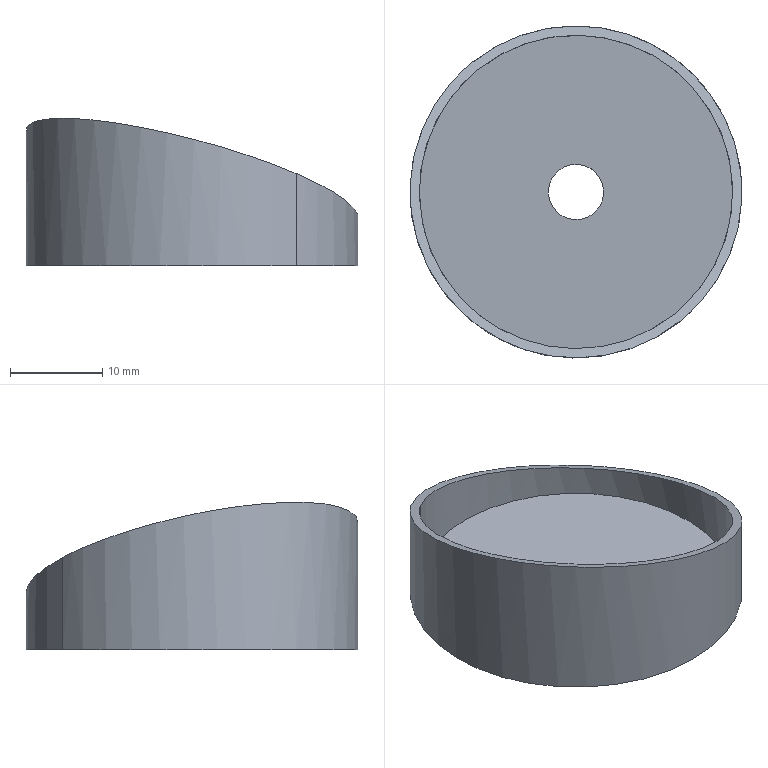Component | SolidWorks | GRingCam-8 | 1 solid | 9 faces | box 36 x 36 x 16 mm | volume 1979 mm3 | cylinder 6 | plane 3 | commonest cylinder face diameters 6 x2 36 x2 34 x2
build123d program:
from build123d import *

# Parameters (mm, degrees)
SKETCH2_R           = 18
SKETCH2_R_2         = 17
BOSS_EXTRUDE1_DEPTH = 8
CUT_EXTRUDE1_DEPTH  = 27
BOSS_EXTRUDE2_START = -1
SKETCH4_R           = 18
SKETCH4_R_2         = 3
BOSS_EXTRUDE2_DEPTH = 1


with BuildPart() as part:
    # Sketch2 → Boss-Extrude1 (new, symmetric)
    with BuildSketch(Plane(origin=(0, 0, 0), x_dir=(1, 0, 0), z_dir=(0, 1, 0))):
        with Locations(Location((0, 0, 0), (0, 0, 270))):
            Circle(SKETCH2_R)
        with Locations(Location((0, 0, 0), (0, 0, 270))):
            Circle(SKETCH2_R_2, mode=Mode.SUBTRACT)
    extrude(amount=BOSS_EXTRUDE1_DEPTH, both=True)

    # Sketch3 → Cut-Extrude1 (cut, symmetric)
    with BuildSketch(Plane.XY):
        Polygon((-24.457, 9.582), (-18, -4), (18, 8), align=None)
    extrude(amount=CUT_EXTRUDE1_DEPTH, both=True, mode=Mode.SUBTRACT)

    # Sketch4 → Boss-Extrude2 (add)
    with BuildSketch(Plane.XZ.offset(8).offset(BOSS_EXTRUDE2_START)):
        with Locations(Location((0, 0, 0), (0, 0, 180))):
            Circle(SKETCH4_R)
        with Locations(Location((0, 0, 0), (0, 0, 270))):
            Circle(SKETCH4_R_2, mode=Mode.SUBTRACT)
    extrude(amount=BOSS_EXTRUDE2_DEPTH)


solid = part.part

# Placed as in the assembly
solid = solid.moved(Location((-15.928, -22.2, 125), (-90, -38.823, 179.998)))
STEP:
#1=COLOUR_RGB('',0.7922,0.8196,0.9333);
#2=FILL_AREA_STYLE_COLOUR('',#1);
#3=FILL_AREA_STYLE('',(#2));
#4=SURFACE_STYLE_FILL_AREA(#3);
#5=SURFACE_SIDE_STYLE('',(#4));
#6=SURFACE_STYLE_USAGE(.BOTH.,#5);
#7=PRESENTATION_STYLE_ASSIGNMENT((#6));
#8=CARTESIAN_POINT('',(-0.7011,-0.782,4.646));
#9=VERTEX_POINT('',#8);
#10=CARTESIAN_POINT('',(-0.553,-0.966,4.646));
#11=VERTEX_POINT('',#10);
#12=CARTESIAN_POINT('',(-0.6271,-0.874,4.646));
#13=DIRECTION('',(0.,0.,-1.));
#14=DIRECTION('',(0.6269,-0.7791,0.));
#15=AXIS2_PLACEMENT_3D('',#12,#13,#14);
#16=CIRCLE('',#15,0.1181);
#17=EDGE_CURVE('',#9,#11,#16,.T.);
#18=ORIENTED_EDGE('',*,*,#17,.F.);
#19=CARTESIAN_POINT('',(-0.7011,-0.782,4.606));
#20=VERTEX_POINT('',#19);
#21=CARTESIAN_POINT('',(-0.7011,-0.782,4.646));
#22=DIRECTION('',(0.,0.,-1.));
#23=VECTOR('',#22,39.37);
#24=LINE('',#21,#23);
#25=EDGE_CURVE('',#9,#20,#24,.T.);
#26=ORIENTED_EDGE('',*,*,#25,.T.);
#27=CARTESIAN_POINT('',(-0.553,-0.966,4.606));
#28=VERTEX_POINT('',#27);
#29=CARTESIAN_POINT('',(-0.6271,-0.874,4.606));
#30=DIRECTION('',(0.,0.,-1.));
#31=DIRECTION('',(0.6269,-0.7791,0.));
#32=AXIS2_PLACEMENT_3D('',#29,#30,#31);
#33=CIRCLE('',#32,0.1181);
#34=EDGE_CURVE('',#20,#28,#33,.T.);
#35=ORIENTED_EDGE('',*,*,#34,.T.);
#36=CARTESIAN_POINT('',(-0.553,-0.966,4.646));
#37=DIRECTION('',(0.,0.,-1.));
#38=VECTOR('',#37,39.37);
#39=LINE('',#36,#38);
#40=EDGE_CURVE('',#11,#28,#39,.T.);
#41=ORIENTED_EDGE('',*,*,#40,.F.);
#42=EDGE_LOOP('',(#18,#26,#35,#41));
#43=FACE_OUTER_BOUND('',#42,.T.);
#44=CARTESIAN_POINT('',(-0.6271,-0.874,4.646));
#45=DIRECTION('',(0.,0.,-1.));
#46=DIRECTION('',(0.6269,-0.7791,0.));
#47=AXIS2_PLACEMENT_3D('',#44,#45,#46);
#48=CYLINDRICAL_SURFACE('',#47,0.1181);
#49=ADVANCED_FACE('',(#43),#48,.F.);
#50=CARTESIAN_POINT('',(-0.1828,-1.426,5.));
#51=VERTEX_POINT('',#50);
#52=CARTESIAN_POINT('',(-1.071,-0.3219,5.));
#53=VERTEX_POINT('',#52);
#54=CARTESIAN_POINT('',(-0.1828,-1.426,5.));
#55=CARTESIAN_POINT('',(-1.287,-2.315,5.472));
#56=CARTESIAN_POINT('',(-2.176,-1.21,5.472));
#57=CARTESIAN_POINT('',(-1.071,-0.3219,5.));
#58=(BOUNDED_CURVE()B_SPLINE_CURVE(3,(#54,#55,#56,#57),.UNSPECIFIED.,.F.,.T.)B_SPLINE_CURVE_WITH_KNOTS((4,4),(1.571,4.712),.UNSPECIFIED.)CURVE()GEOMETRIC_REPRESENTATION_ITEM()RATIONAL_B_SPLINE_CURVE((1.,0.3333,0.3333,1.))REPRESENTATION_ITEM(''));
#59=EDGE_CURVE('',#51,#53,#58,.T.);
#60=ORIENTED_EDGE('',*,*,#59,.T.);
#61=CARTESIAN_POINT('',(-1.071,-0.3219,4.606));
#62=VERTEX_POINT('',#61);
#63=CARTESIAN_POINT('',(-1.071,-0.3219,5.236));
#64=DIRECTION('',(0.,0.,-1.));
#65=VECTOR('',#64,39.37);
#66=LINE('',#63,#65);
#67=EDGE_CURVE('',#53,#62,#66,.T.);
#68=ORIENTED_EDGE('',*,*,#67,.T.);
#69=CARTESIAN_POINT('',(-0.1828,-1.426,4.606));
#70=VERTEX_POINT('',#69);
#71=CARTESIAN_POINT('',(-0.6271,-0.874,4.606));
#72=DIRECTION('',(-0.,-0.,1.));
#73=DIRECTION('',(-0.6269,0.7791,0.));
#74=AXIS2_PLACEMENT_3D('',#71,#72,#73);
#75=CIRCLE('',#74,0.7087);
#76=EDGE_CURVE('',#62,#70,#75,.T.);
#77=ORIENTED_EDGE('',*,*,#76,.T.);
#78=CARTESIAN_POINT('',(-0.1828,-1.426,5.236));
#79=DIRECTION('',(0.,0.,-1.));
#80=VECTOR('',#79,39.37);
#81=LINE('',#78,#80);
#82=EDGE_CURVE('',#51,#70,#81,.T.);
#83=ORIENTED_EDGE('',*,*,#82,.F.);
#84=EDGE_LOOP('',(#60,#68,#77,#83));
#85=FACE_OUTER_BOUND('',#84,.T.);
#86=CARTESIAN_POINT('',(-0.6271,-0.874,5.236));
#87=DIRECTION('',(0.,0.,-1.));
#88=DIRECTION('',(0.6269,-0.7791,0.));
#89=AXIS2_PLACEMENT_3D('',#86,#87,#88);
#90=CYLINDRICAL_SURFACE('',#89,0.7087);
#91=ADVANCED_FACE('',(#85),#90,.T.);
#92=CARTESIAN_POINT('',(-1.047,-0.3526,5.));
#93=VERTEX_POINT('',#92);
#94=CARTESIAN_POINT('',(-0.2075,-1.395,5.));
#95=VERTEX_POINT('',#94);
#96=CARTESIAN_POINT('',(-1.047,-0.3526,5.));
#97=CARTESIAN_POINT('',(-0.003795,0.4866,4.554));
#98=CARTESIAN_POINT('',(0.8354,-0.5563,4.554));
#99=CARTESIAN_POINT('',(-0.2075,-1.395,5.));
#100=(BOUNDED_CURVE()B_SPLINE_CURVE(3,(#96,#97,#98,#99),.UNSPECIFIED.,.F.,.F.)B_SPLINE_CURVE_WITH_KNOTS((4,4),(4.712,7.854),.UNSPECIFIED.)CURVE()GEOMETRIC_REPRESENTATION_ITEM()RATIONAL_B_SPLINE_CURVE((1.,0.3333,0.3333,1.))REPRESENTATION_ITEM(''));
#101=EDGE_CURVE('',#93,#95,#100,.T.);
#102=ORIENTED_EDGE('',*,*,#101,.F.);
#103=CARTESIAN_POINT('',(-1.047,-0.3526,4.646));
#104=VERTEX_POINT('',#103);
#105=CARTESIAN_POINT('',(-1.047,-0.3526,5.236));
#106=DIRECTION('',(0.,0.,-1.));
#107=VECTOR('',#106,39.37);
#108=LINE('',#105,#107);
#109=EDGE_CURVE('',#93,#104,#108,.T.);
#110=ORIENTED_EDGE('',*,*,#109,.T.);
#111=CARTESIAN_POINT('',(-0.2075,-1.395,4.646));
#112=VERTEX_POINT('',#111);
#113=CARTESIAN_POINT('',(-0.6271,-0.874,4.646));
#114=DIRECTION('',(0.,0.,-1.));
#115=DIRECTION('',(0.6269,-0.7791,0.));
#116=AXIS2_PLACEMENT_3D('',#113,#114,#115);
#117=CIRCLE('',#116,0.6693);
#118=EDGE_CURVE('',#104,#112,#117,.T.);
#119=ORIENTED_EDGE('',*,*,#118,.T.);
#120=CARTESIAN_POINT('',(-0.2075,-1.395,5.236));
#121=DIRECTION('',(0.,0.,-1.));
#122=VECTOR('',#121,39.37);
#123=LINE('',#120,#122);
#124=EDGE_CURVE('',#95,#112,#123,.T.);
#125=ORIENTED_EDGE('',*,*,#124,.F.);
#126=EDGE_LOOP('',(#102,#110,#119,#125));
#127=FACE_OUTER_BOUND('',#126,.T.);
#128=CARTESIAN_POINT('',(-0.6271,-0.874,5.236));
#129=DIRECTION('',(0.,0.,-1.));
#130=DIRECTION('',(0.6269,-0.7791,0.));
#131=AXIS2_PLACEMENT_3D('',#128,#129,#130);
#132=CYLINDRICAL_SURFACE('',#131,0.6693);
#133=ADVANCED_FACE('',(#127),#132,.F.);
#134=ORIENTED_EDGE('',*,*,#109,.F.);
#135=CARTESIAN_POINT('',(-0.2075,-1.395,5.));
#136=CARTESIAN_POINT('',(-1.25,-2.235,5.446));
#137=CARTESIAN_POINT('',(-2.09,-1.192,5.446));
#138=CARTESIAN_POINT('',(-1.047,-0.3526,5.));
#139=(BOUNDED_CURVE()B_SPLINE_CURVE(3,(#135,#136,#137,#138),.UNSPECIFIED.,.F.,.T.)B_SPLINE_CURVE_WITH_KNOTS((4,4),(1.571,4.712),.UNSPECIFIED.)CURVE()GEOMETRIC_REPRESENTATION_ITEM()RATIONAL_B_SPLINE_CURVE((1.,0.3333,0.3333,1.))REPRESENTATION_ITEM(''));
#140=EDGE_CURVE('',#95,#93,#139,.T.);
#141=ORIENTED_EDGE('',*,*,#140,.F.);
#142=ORIENTED_EDGE('',*,*,#124,.T.);
#143=CARTESIAN_POINT('',(-0.6271,-0.874,4.646));
#144=DIRECTION('',(0.,0.,-1.));
#145=DIRECTION('',(0.6269,-0.7791,0.));
#146=AXIS2_PLACEMENT_3D('',#143,#144,#145);
#147=CIRCLE('',#146,0.6693);
#148=EDGE_CURVE('',#112,#104,#147,.T.);
#149=ORIENTED_EDGE('',*,*,#148,.T.);
#150=EDGE_LOOP('',(#134,#141,#142,#149));
#151=FACE_OUTER_BOUND('',#150,.T.);
#152=CARTESIAN_POINT('',(-0.6271,-0.874,5.236));
#153=DIRECTION('',(0.,0.,-1.));
#154=DIRECTION('',(0.6269,-0.7791,0.));
#155=AXIS2_PLACEMENT_3D('',#152,#153,#154);
#156=CYLINDRICAL_SURFACE('',#155,0.6693);
#157=ADVANCED_FACE('',(#151),#156,.F.);
#158=CARTESIAN_POINT('',(-0.6271,-0.874,4.606));
#159=DIRECTION('',(-0.,-0.,1.));
#160=DIRECTION('',(-0.6269,0.7791,0.));
#161=AXIS2_PLACEMENT_3D('',#158,#159,#160);
#162=CIRCLE('',#161,0.7087);
#163=EDGE_CURVE('',#70,#62,#162,.T.);
#164=ORIENTED_EDGE('',*,*,#163,.F.);
#165=ORIENTED_EDGE('',*,*,#76,.F.);
#166=EDGE_LOOP('',(#164,#165));
#167=FACE_OUTER_BOUND('',#166,.T.);
#168=CARTESIAN_POINT('',(-0.6271,-0.874,4.606));
#169=DIRECTION('',(0.,0.,-1.));
#170=DIRECTION('',(0.6269,-0.7791,0.));
#171=AXIS2_PLACEMENT_3D('',#168,#169,#170);
#172=CIRCLE('',#171,0.1181);
#173=EDGE_CURVE('',#28,#20,#172,.T.);
#174=ORIENTED_EDGE('',*,*,#173,.F.);
#175=ORIENTED_EDGE('',*,*,#34,.F.);
#176=EDGE_LOOP('',(#174,#175));
#177=FACE_BOUND('',#176,.T.);
#178=CARTESIAN_POINT('',(-0.6271,-0.874,4.606));
#179=DIRECTION('',(-0.,-0.,1.));
#180=DIRECTION('',(-0.6269,0.7791,0.));
#181=AXIS2_PLACEMENT_3D('',#178,#179,#180);
#182=PLANE('',#181);
#183=ADVANCED_FACE('',(#167,#177),#182,.F.);
#184=ORIENTED_EDGE('',*,*,#67,.F.);
#185=CARTESIAN_POINT('',(-1.071,-0.3219,5.));
#186=CARTESIAN_POINT('',(0.03287,0.5666,4.528));
#187=CARTESIAN_POINT('',(0.9214,-0.5376,4.528));
#188=CARTESIAN_POINT('',(-0.1828,-1.426,5.));
#189=(BOUNDED_CURVE()B_SPLINE_CURVE(3,(#185,#186,#187,#188),.UNSPECIFIED.,.F.,.F.)B_SPLINE_CURVE_WITH_KNOTS((4,4),(4.712,7.854),.UNSPECIFIED.)CURVE()GEOMETRIC_REPRESENTATION_ITEM()RATIONAL_B_SPLINE_CURVE((1.,0.3333,0.3333,1.))REPRESENTATION_ITEM(''));
#190=EDGE_CURVE('',#53,#51,#189,.T.);
#191=ORIENTED_EDGE('',*,*,#190,.T.);
#192=ORIENTED_EDGE('',*,*,#82,.T.);
#193=ORIENTED_EDGE('',*,*,#163,.T.);
#194=EDGE_LOOP('',(#184,#191,#192,#193));
#195=FACE_OUTER_BOUND('',#194,.T.);
#196=CARTESIAN_POINT('',(-0.6271,-0.874,5.236));
#197=DIRECTION('',(0.,0.,-1.));
#198=DIRECTION('',(0.6269,-0.7791,0.));
#199=AXIS2_PLACEMENT_3D('',#196,#197,#198);
#200=CYLINDRICAL_SURFACE('',#199,0.7087);
#201=ADVANCED_FACE('',(#195),#200,.T.);
#202=ORIENTED_EDGE('',*,*,#140,.T.);
#203=ORIENTED_EDGE('',*,*,#101,.T.);
#204=EDGE_LOOP('',(#202,#203));
#205=FACE_BOUND('',#204,.T.);
#206=ORIENTED_EDGE('',*,*,#59,.F.);
#207=ORIENTED_EDGE('',*,*,#190,.F.);
#208=EDGE_LOOP('',(#206,#207));
#209=FACE_OUTER_BOUND('',#208,.T.);
#210=CARTESIAN_POINT('',(0.5914,-1.258,4.764));
#211=DIRECTION('',(-0.2464,-0.1982,-0.9487));
#212=DIRECTION('',(-0.7391,-0.5947,0.3162));
#213=AXIS2_PLACEMENT_3D('',#210,#211,#212);
#214=PLANE('',#213);
#215=ADVANCED_FACE('',(#205,#209),#214,.F.);
#216=ORIENTED_EDGE('',*,*,#148,.F.);
#217=ORIENTED_EDGE('',*,*,#118,.F.);
#218=EDGE_LOOP('',(#216,#217));
#219=FACE_OUTER_BOUND('',#218,.T.);
#220=CARTESIAN_POINT('',(-0.6271,-0.874,4.646));
#221=DIRECTION('',(0.,0.,-1.));
#222=DIRECTION('',(0.6269,-0.7791,0.));
#223=AXIS2_PLACEMENT_3D('',#220,#221,#222);
#224=CIRCLE('',#223,0.1181);
#225=EDGE_CURVE('',#11,#9,#224,.T.);
#226=ORIENTED_EDGE('',*,*,#225,.T.);
#227=ORIENTED_EDGE('',*,*,#17,.T.);
#228=EDGE_LOOP('',(#226,#227));
#229=FACE_BOUND('',#228,.T.);
#230=CARTESIAN_POINT('',(-0.6271,-0.874,4.646));
#231=DIRECTION('',(0.,0.,-1.));
#232=DIRECTION('',(0.6269,-0.7791,-0.));
#233=AXIS2_PLACEMENT_3D('',#230,#231,#232);
#234=PLANE('',#233);
#235=ADVANCED_FACE('',(#219,#229),#234,.F.);
#236=ORIENTED_EDGE('',*,*,#25,.F.);
#237=ORIENTED_EDGE('',*,*,#225,.F.);
#238=ORIENTED_EDGE('',*,*,#40,.T.);
#239=ORIENTED_EDGE('',*,*,#173,.T.);
#240=EDGE_LOOP('',(#236,#237,#238,#239));
#241=FACE_OUTER_BOUND('',#240,.T.);
#242=CARTESIAN_POINT('',(-0.6271,-0.874,4.646));
#243=DIRECTION('',(0.,0.,-1.));
#244=DIRECTION('',(0.6269,-0.7791,0.));
#245=AXIS2_PLACEMENT_3D('',#242,#243,#244);
#246=CYLINDRICAL_SURFACE('',#245,0.1181);
#247=ADVANCED_FACE('',(#241),#246,.F.);
#248=CLOSED_SHELL('',(#49,#91,#133,#157,#183,#201,#215,#235,#247));
#249=MANIFOLD_SOLID_BREP('',#248);
#250=STYLED_ITEM('',(#7),#249);
#251=(LENGTH_UNIT()NAMED_UNIT(*)SI_UNIT($,.METRE.));
#252=LENGTH_MEASURE_WITH_UNIT(LENGTH_MEASURE(0.0254),#251);
#253=DIMENSIONAL_EXPONENTS(1.,0.,0.,0.,0.,0.,0.);
#254=(CONVERSION_BASED_UNIT('',#252)LENGTH_UNIT()NAMED_UNIT(#253));
#255=UNCERTAINTY_MEASURE_WITH_UNIT(LENGTH_MEASURE(0.00001),#254,'','');
#256=(NAMED_UNIT(*)PLANE_ANGLE_UNIT()SI_UNIT($,.RADIAN.));
#257=(NAMED_UNIT(*)SI_UNIT($,.STERADIAN.)SOLID_ANGLE_UNIT());
#258=(GEOMETRIC_REPRESENTATION_CONTEXT(3)GLOBAL_UNCERTAINTY_ASSIGNED_CONTEXT((#255))GLOBAL_UNIT_ASSIGNED_CONTEXT((#254,#256,#257))REPRESENTATION_CONTEXT('',''));
#259=MECHANICAL_DESIGN_GEOMETRIC_PRESENTATION_REPRESENTATION('',(#250),#258);
#260=CARTESIAN_POINT('',(0.,0.,0.));
#261=DIRECTION('',(0.,0.,1.));
#262=DIRECTION('',(1.,0.,0.));
#263=AXIS2_PLACEMENT_3D('',#260,#261,#262);
#264=(LENGTH_UNIT()NAMED_UNIT(*)SI_UNIT($,.METRE.));
#265=LENGTH_MEASURE_WITH_UNIT(LENGTH_MEASURE(0.0254),#264);
#266=DIMENSIONAL_EXPONENTS(1.,0.,0.,0.,0.,0.,0.);
#267=(CONVERSION_BASED_UNIT('',#265)LENGTH_UNIT()NAMED_UNIT(#266));
#268=UNCERTAINTY_MEASURE_WITH_UNIT(LENGTH_MEASURE(0.00001),#267,'','');
#269=(NAMED_UNIT(*)PLANE_ANGLE_UNIT()SI_UNIT($,.RADIAN.));
#270=(NAMED_UNIT(*)SI_UNIT($,.STERADIAN.)SOLID_ANGLE_UNIT());
#271=(GEOMETRIC_REPRESENTATION_CONTEXT(3)GLOBAL_UNCERTAINTY_ASSIGNED_CONTEXT((#268))GLOBAL_UNIT_ASSIGNED_CONTEXT((#267,#269,#270))REPRESENTATION_CONTEXT('',''));
#272=ADVANCED_BREP_SHAPE_REPRESENTATION('',(#249,#263),#271);
#273=PRESENTATION_LAYER_ASSIGNMENT('','',(#250));